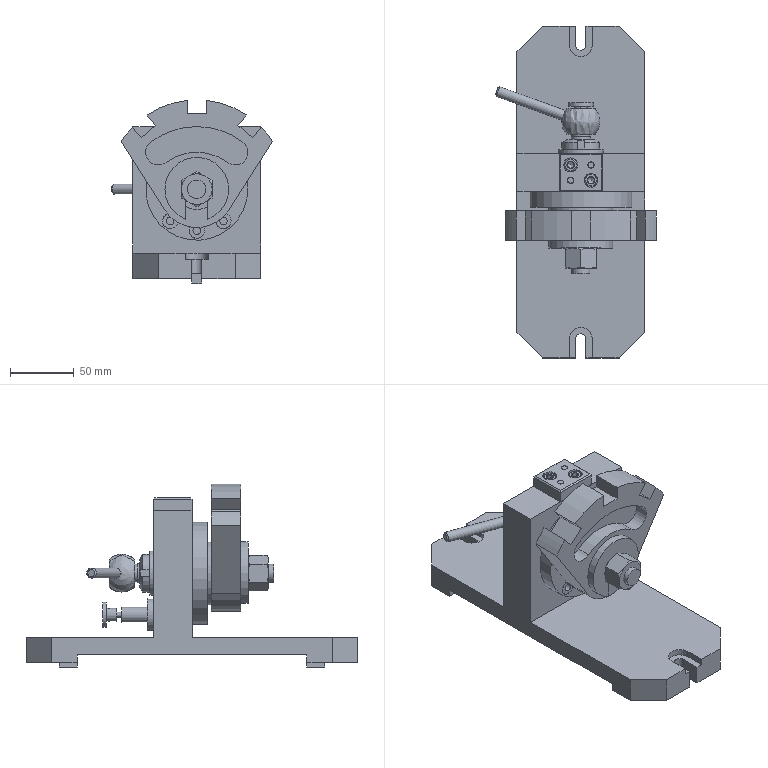Assembly | NX | mm | 29 component files | 29 solids | 487 faces | box 126.09 x 260 x 143.6 mm | volume 948178 mm3 | plane 273 | cylinder 103 | cone 91 | torus 14 | spline 5 | sphere 1 | commonest cylinder face diameters 12 x9 1.886 x6 5 x6 20 x5 2.874 x4 5.795 x4 1.5 x4 140 x4
Bill of materials:
GB812-88,M16x1_5 | 1 |  | Round Nut, GB 812-88,M16x1_5
unnamed part 1 | 1 |  | Flat fan- or sector-shaped plate with a rounded narrow end, one round through hole near that end, and three rectangular notches cut into the wide arced edge.
GB-T119.1-2000,5x20 | 2 |  | Parallel Pin, GB-T 119.1-2000,5x20
unnamed part 2 | 1 |  | Square block with a chamfer around the top face edges and four round through holes: two larger and two smaller, each pair on opposite diagonals.
GB-T70.1-2000,M3x8 | 2 |  | Hexagon Socket Head Cap Screw, GB-T 70.1-2000,M3x8
unnamed part 3 | 1 |  | Thin circular disc with a U-shaped slot running from the outer edge past the center and ending in a rounded end.
unnamed part 4 | 2 |  | Rectangular block with four parallel long edges chamfered and a single round hole through the center of the top face.
GB-T70.1-2000,M6x10 | 2 |  | Hexagon Socket Head Cap Screw, GB-T 70.1-2000,M6x10
unnamed part 5 | 1 |  | Thick circular disc with a large central through hole and three smaller through holes grouped in an arc on one side.
unnamed part 6 | 1 |  | Stepped cylindrical shaft with a thin large-diameter flange, a larger collar on one side, plain cylindrical sections, and a reduced end section that appears to have a flat.
unnamed part 7 | 1 |  | Hollow cylindrical tube with an integral circular flange part-way along its length; the flange has three small holes evenly spaced around it.
unnamed part 8 | 1 |  | Spherical knob truncated by two parallel flat faces, with a square hole through the flats and a straight cylindrical rod sticking out sideways from the sphere.
unnamed part 9 | 1 |  | Long slender stepped pin with a short end section, a larger cylindrical collar, and a long small-diameter shank with a small cross hole near its far end.
unnamed part 10 | 3 |  | Plain thick-walled cylindrical tube or sleeve, with a length roughly equal to its outer diameter and a concentric through bore.
GB-T70.1-2000,M2x5 | 3 |  | Hexagon Socket Head Cap Screw, GB-T 70.1-2000,M2x5
unnamed part 11 | 1 |  | Thin-walled flanged sleeve: a cylindrical tube with a thin outward flange at one end and a through bore.
unnamed part 12 | 1 |  | Flanged hub: a large circular flange disc with a smaller coaxial cylindrical boss, a central through bore, and a small radial hole through the boss wall.
GB-T41-2000,M16x2 | 1 |  | Hexagonal prism with a central through-bore and chamfered corners at both end faces; shaped like a hex nut.
unnamed part 13 | 1 |  | Helical coil of round-section wire with constant diameter and roughly uniform open pitch, about 7 to 8 turns. It looks like a cylindrical helical spring, and the ends appear to be cut or ground flat.
unnamed part 14 | 1 |  | T-shaped bracket. A rectangular upright block stands at the middle of a long, flat base plate. The base plate has chamfered corners and an open-ended slot at each end. The upright has a large through hole, a smaller hole below it, and four small holes in a 2x2 pattern on its top face.
GB-T119.1-2000,1.5x10 | 1 |  | Parallel Pin, GB-T 119.1-2000,1.5x10
Mates:
1. fix | fixture_body 1 component
2. concentric | locating_mandrel 1 edge | sector_part 1 edge
3. concentric | indexing_plate 1 edge | locating_mandrel 1 edge
4. concentric | C_washer 1 edge | sector_part 1 edge
5. concentric | GB-T41-2000_M16x2 1 edge | C_washer 1 edge
6. concentric | locating_bushing 3 edge | indexing_plate 1 edge
7. bond | indexing_plate 1 component | assembly component
8. bond | locating_bushing 3 component | assembly component
9. bond | locating_bushing 2 component | assembly component
10. bond | locating_bushing 1 component | assembly component
11. circular | assembly datumaxis | assembly cartesiancoordinatesystem | assembly cartesiancoordinatesystem | assembly cartesiancoordinatesystem
12. concentric | bushing 1 edge | fixture_body 1 edge
13. concentric | GB812-88_M16x1_5 1 edge | bushing 1 edge
14. concentric | pin 1 edge | locating_bushing 2 edge
15. concentric | spring 1 edge | pin 1 edge
16. concentric | handle_1 1 edge | pin 1 edge
17. concentric | handle 1 edge | locating_mandrel 1 edge
18. touch align | GB-T119_1-2000_1_5x10 1 face | handle_1 1 face
19. touch align | square_tool_block 1 face | fixture_body 1 face
20. touch align | square_tool_block 1 face | fixture_body 1 face
21. center | square_tool_block 1 face | square_tool_block 1 face | fixture_body 1 face | fixture_body 1 face
22. concentric | indexing_plate 1 edge | fixture_body 1 edge
23. concentric | sleeve 1 edge | fixture_body 1 edge
24. bond | sleeve 1 component | assembly component
25. bond | GB-T70_1-2000_M2x5 3 component | assembly component
26. bond | GB-T70_1-2000_M2x5 2 component | assembly component
27. bond | GB-T70_1-2000_M2x5 1 component | assembly component
28. circular | assembly datumaxis | assembly cartesiancoordinatesystem | assembly cartesiancoordinatesystem | assembly cartesiancoordinatesystem
29. touch align | locating_key 2 face | fixture_body 1 face
30. touch align | locating_key 2 face | fixture_body 1 face
31. touch align | locating_key 2 face | fixture_body 1 face
32. bond | fixture_body 1 component | assembly component
33. bond | locating_key 2 component | assembly component
34. bond | locating_key 1 component | assembly component
35. linear | assembly datumaxis | assembly cartesiancoordinatesystem | assembly cartesiancoordinatesystem
36. bond | GB-T70_1-2000_M3x8 2 component | assembly component
37. bond | GB-T70_1-2000_M3x8 1 component | assembly component
38. linear | assembly datumaxis | assembly cartesiancoordinatesystem | assembly cartesiancoordinatesystem